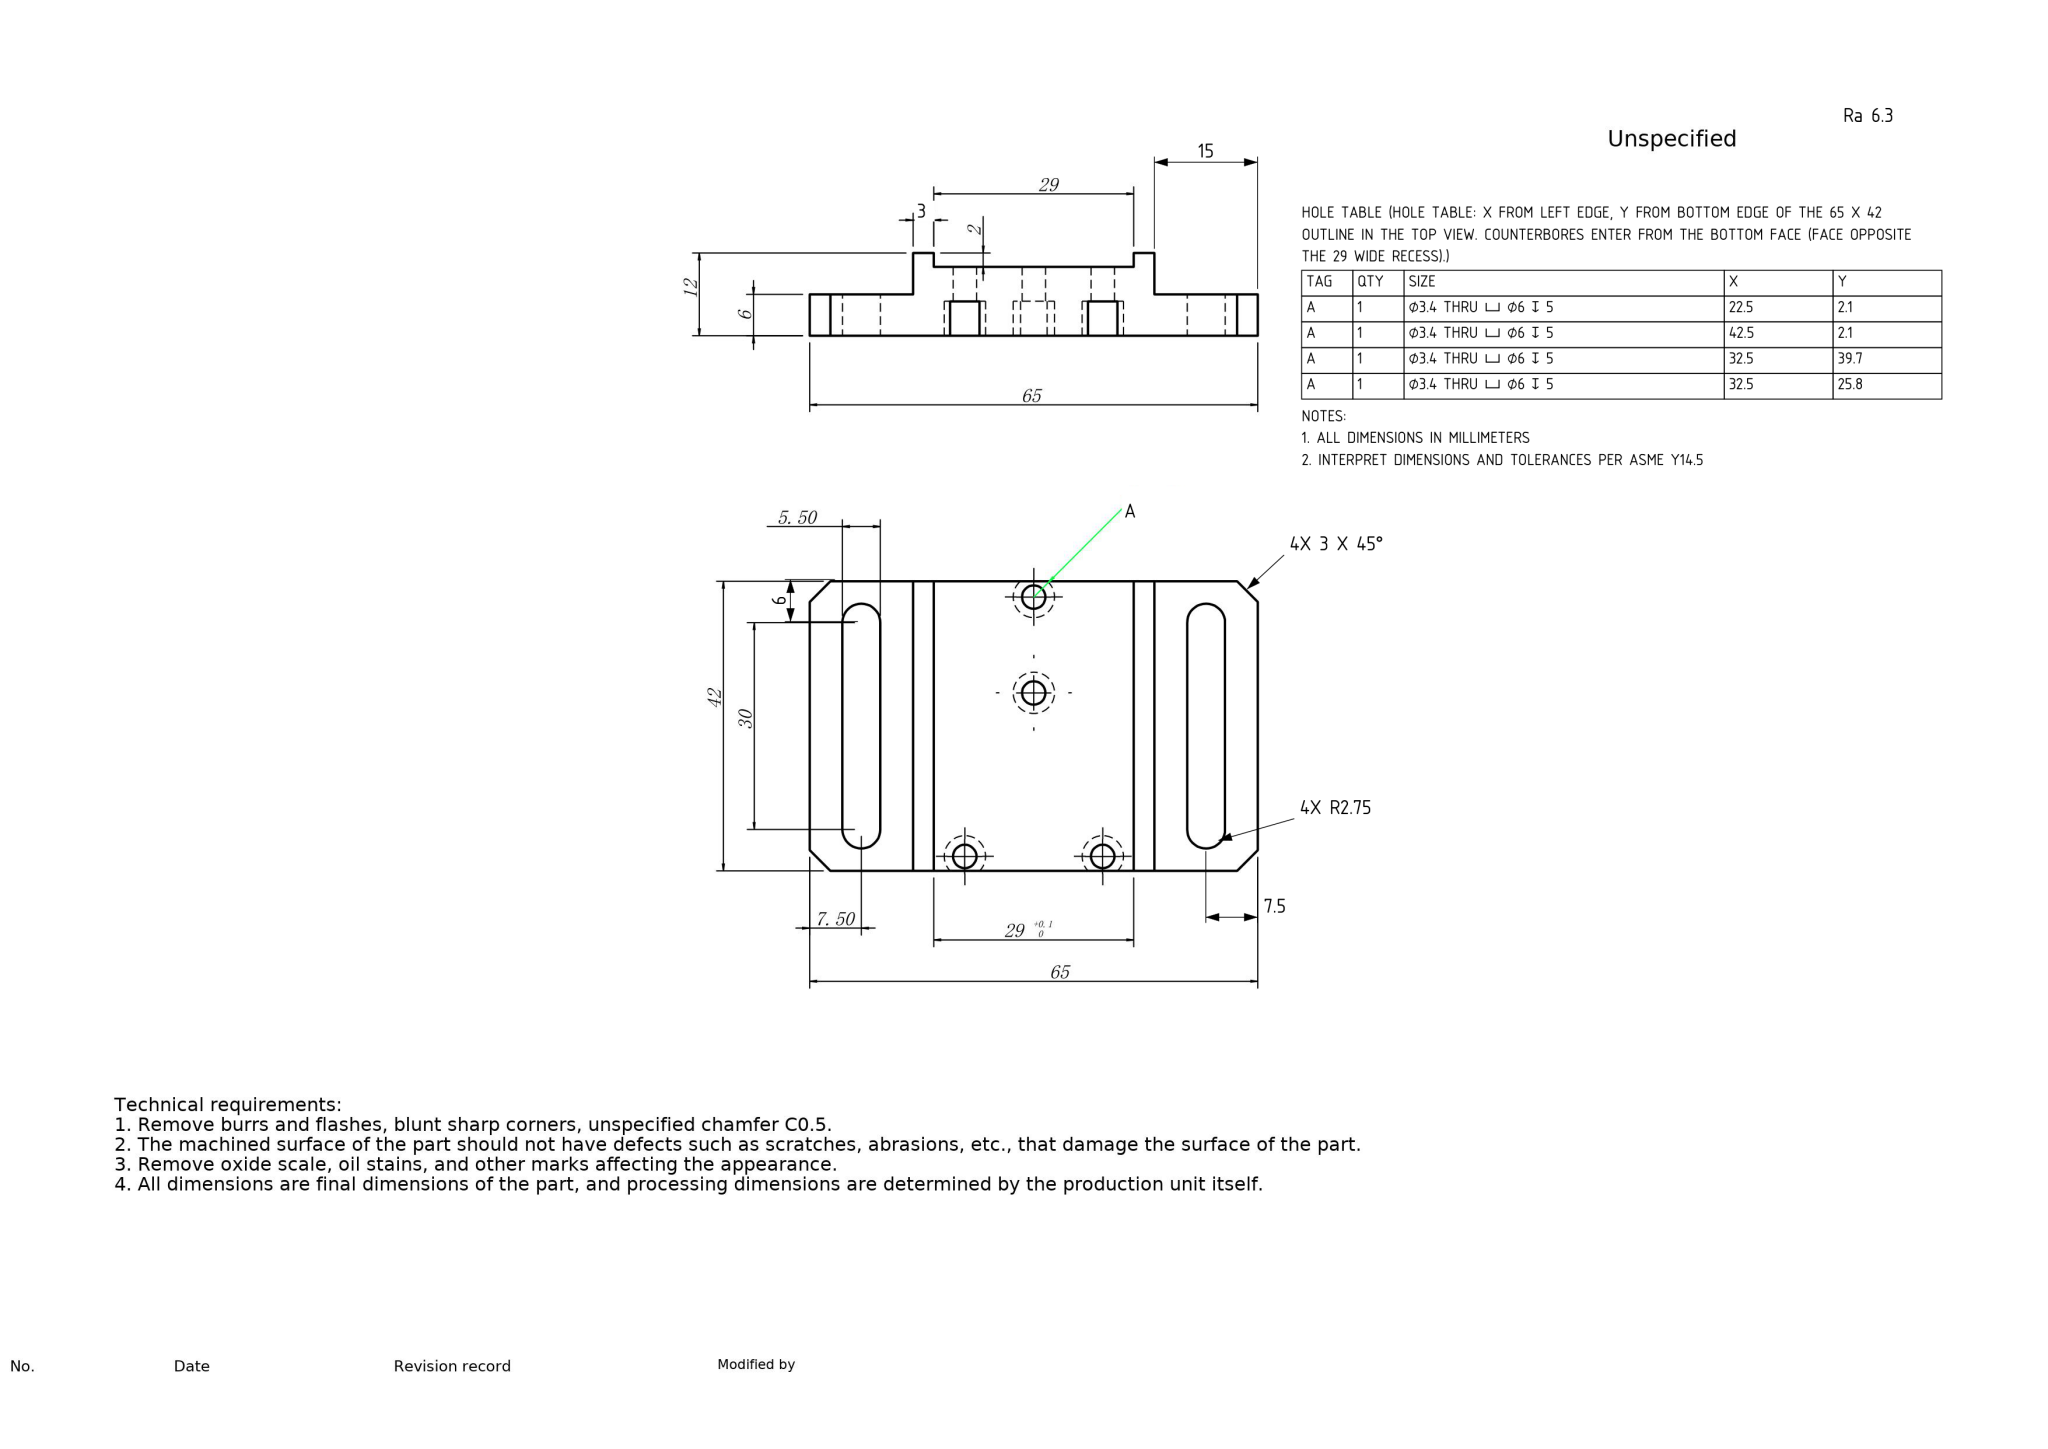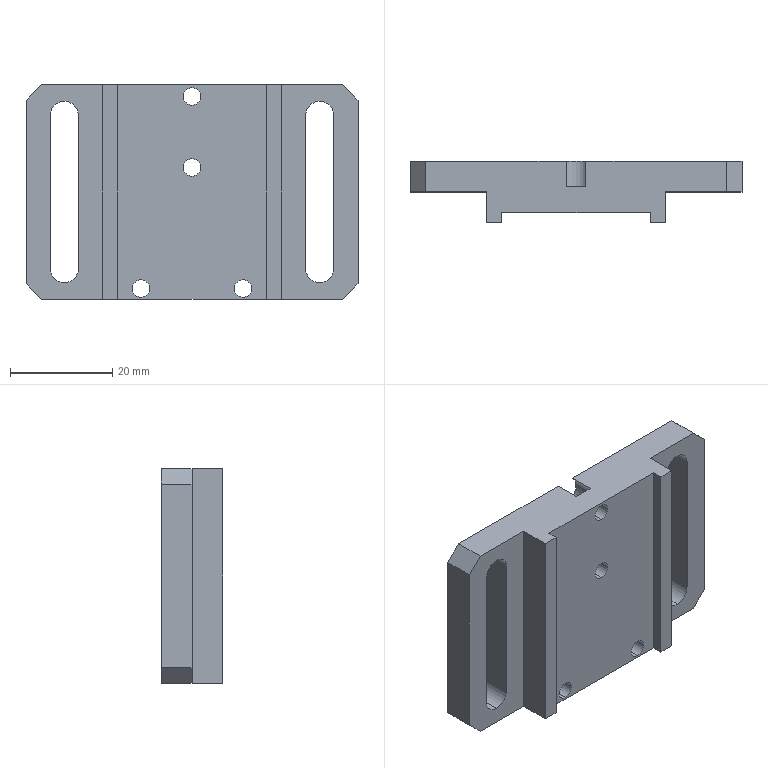Part | NX | mm | 1 solid | 47 faces | box 65 x 12 x 42 mm | volume 19680 mm3 | plane 26 | cylinder 21 | commonest cylinder face diameters 3.4 x8 6 x7 5.5 x6